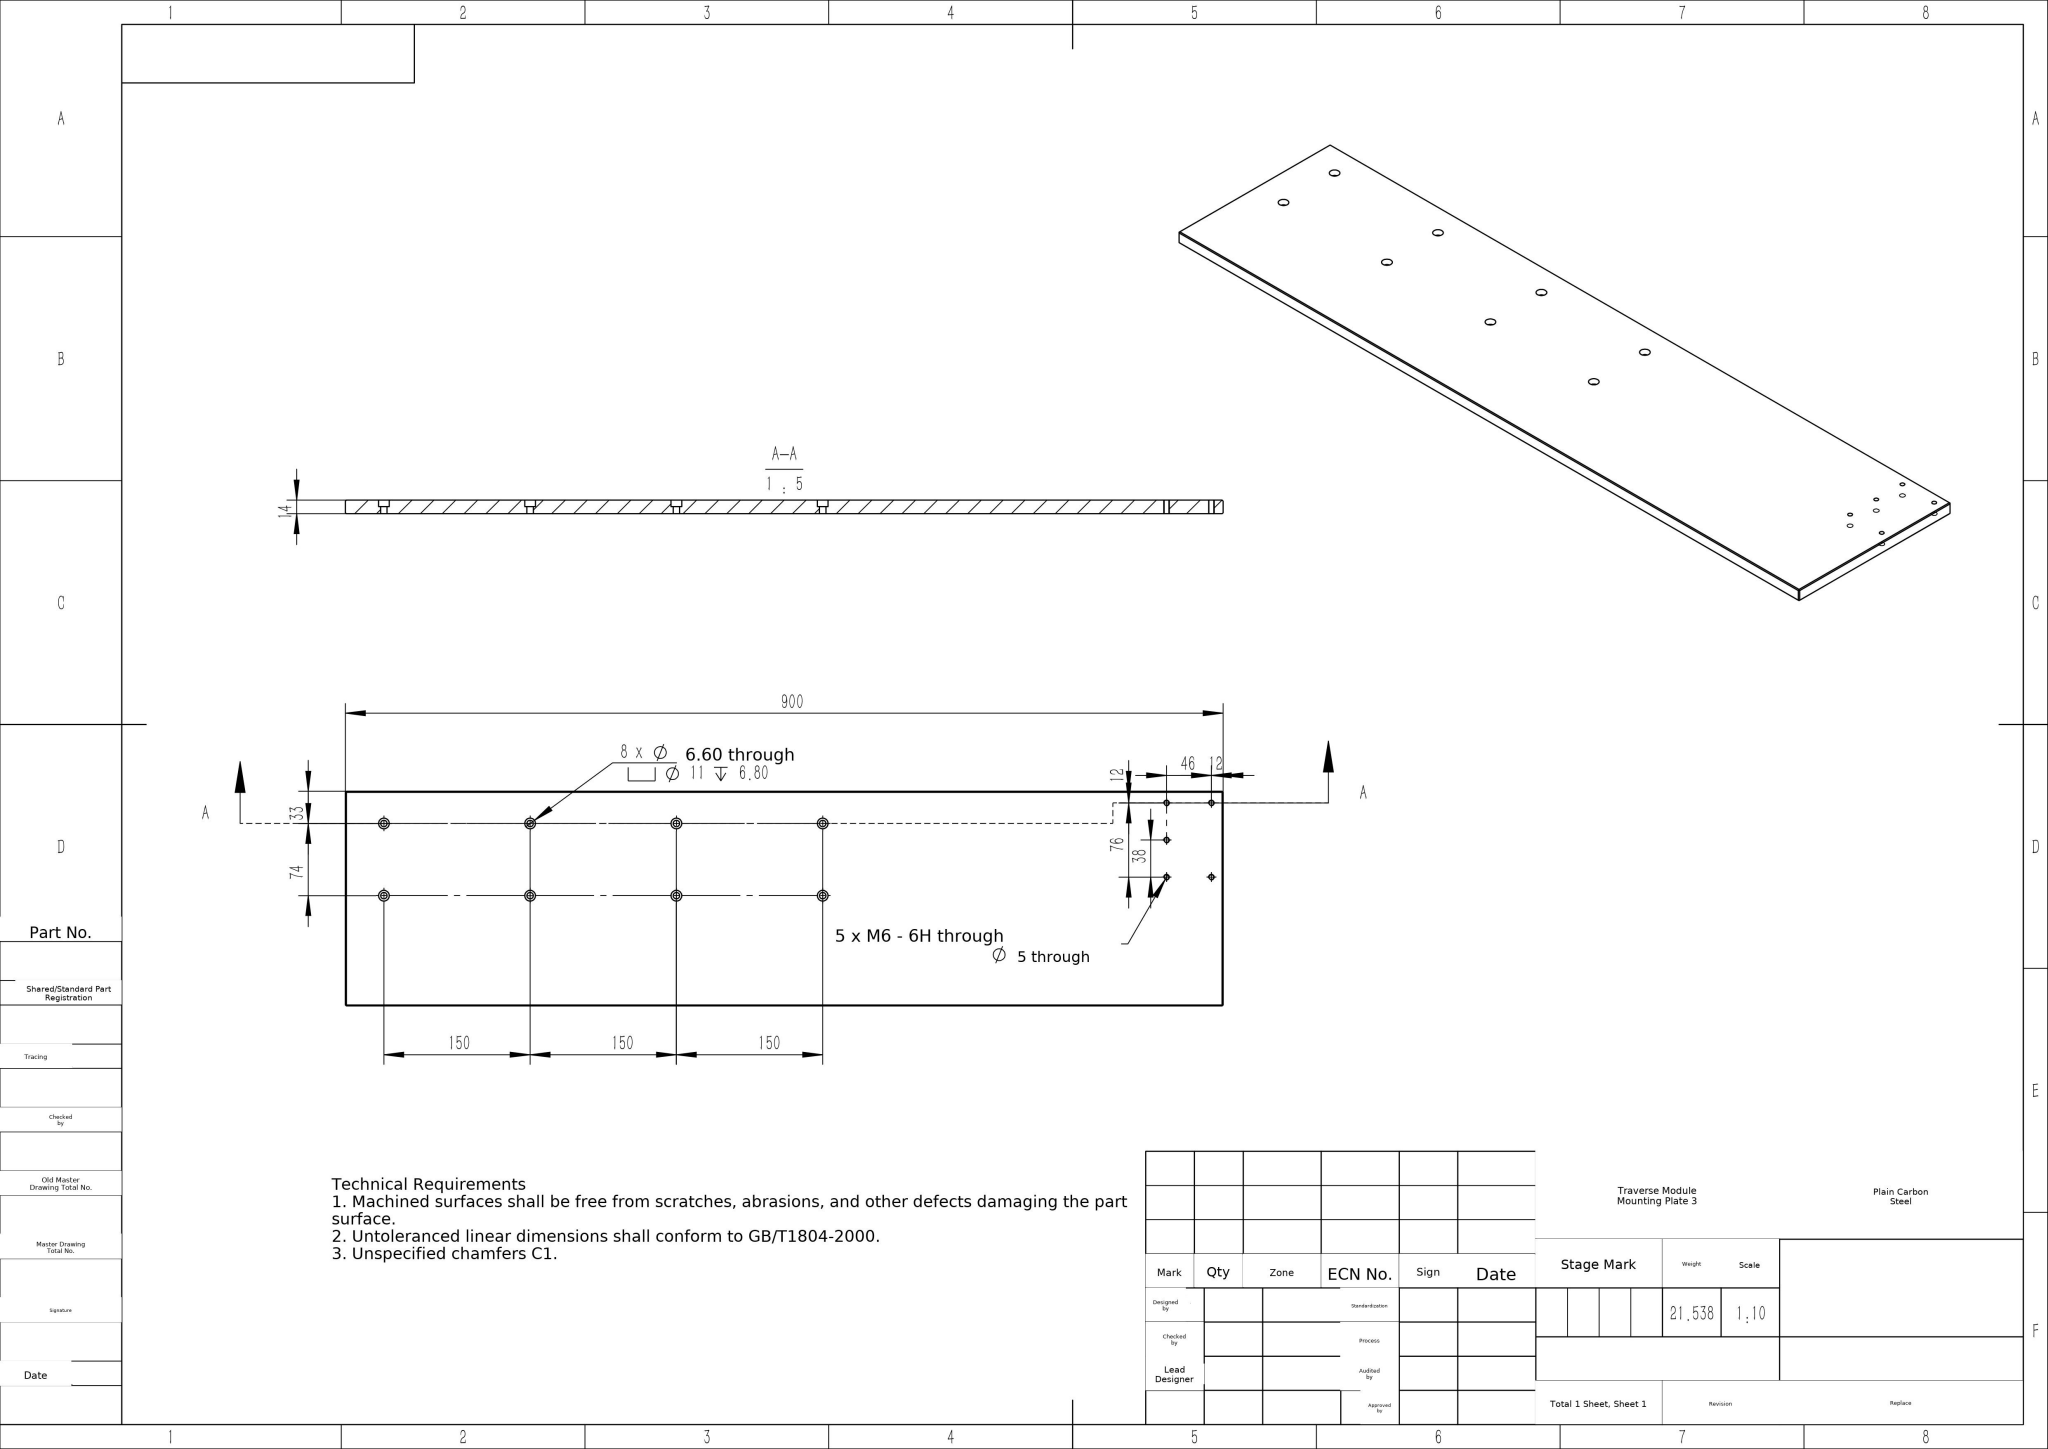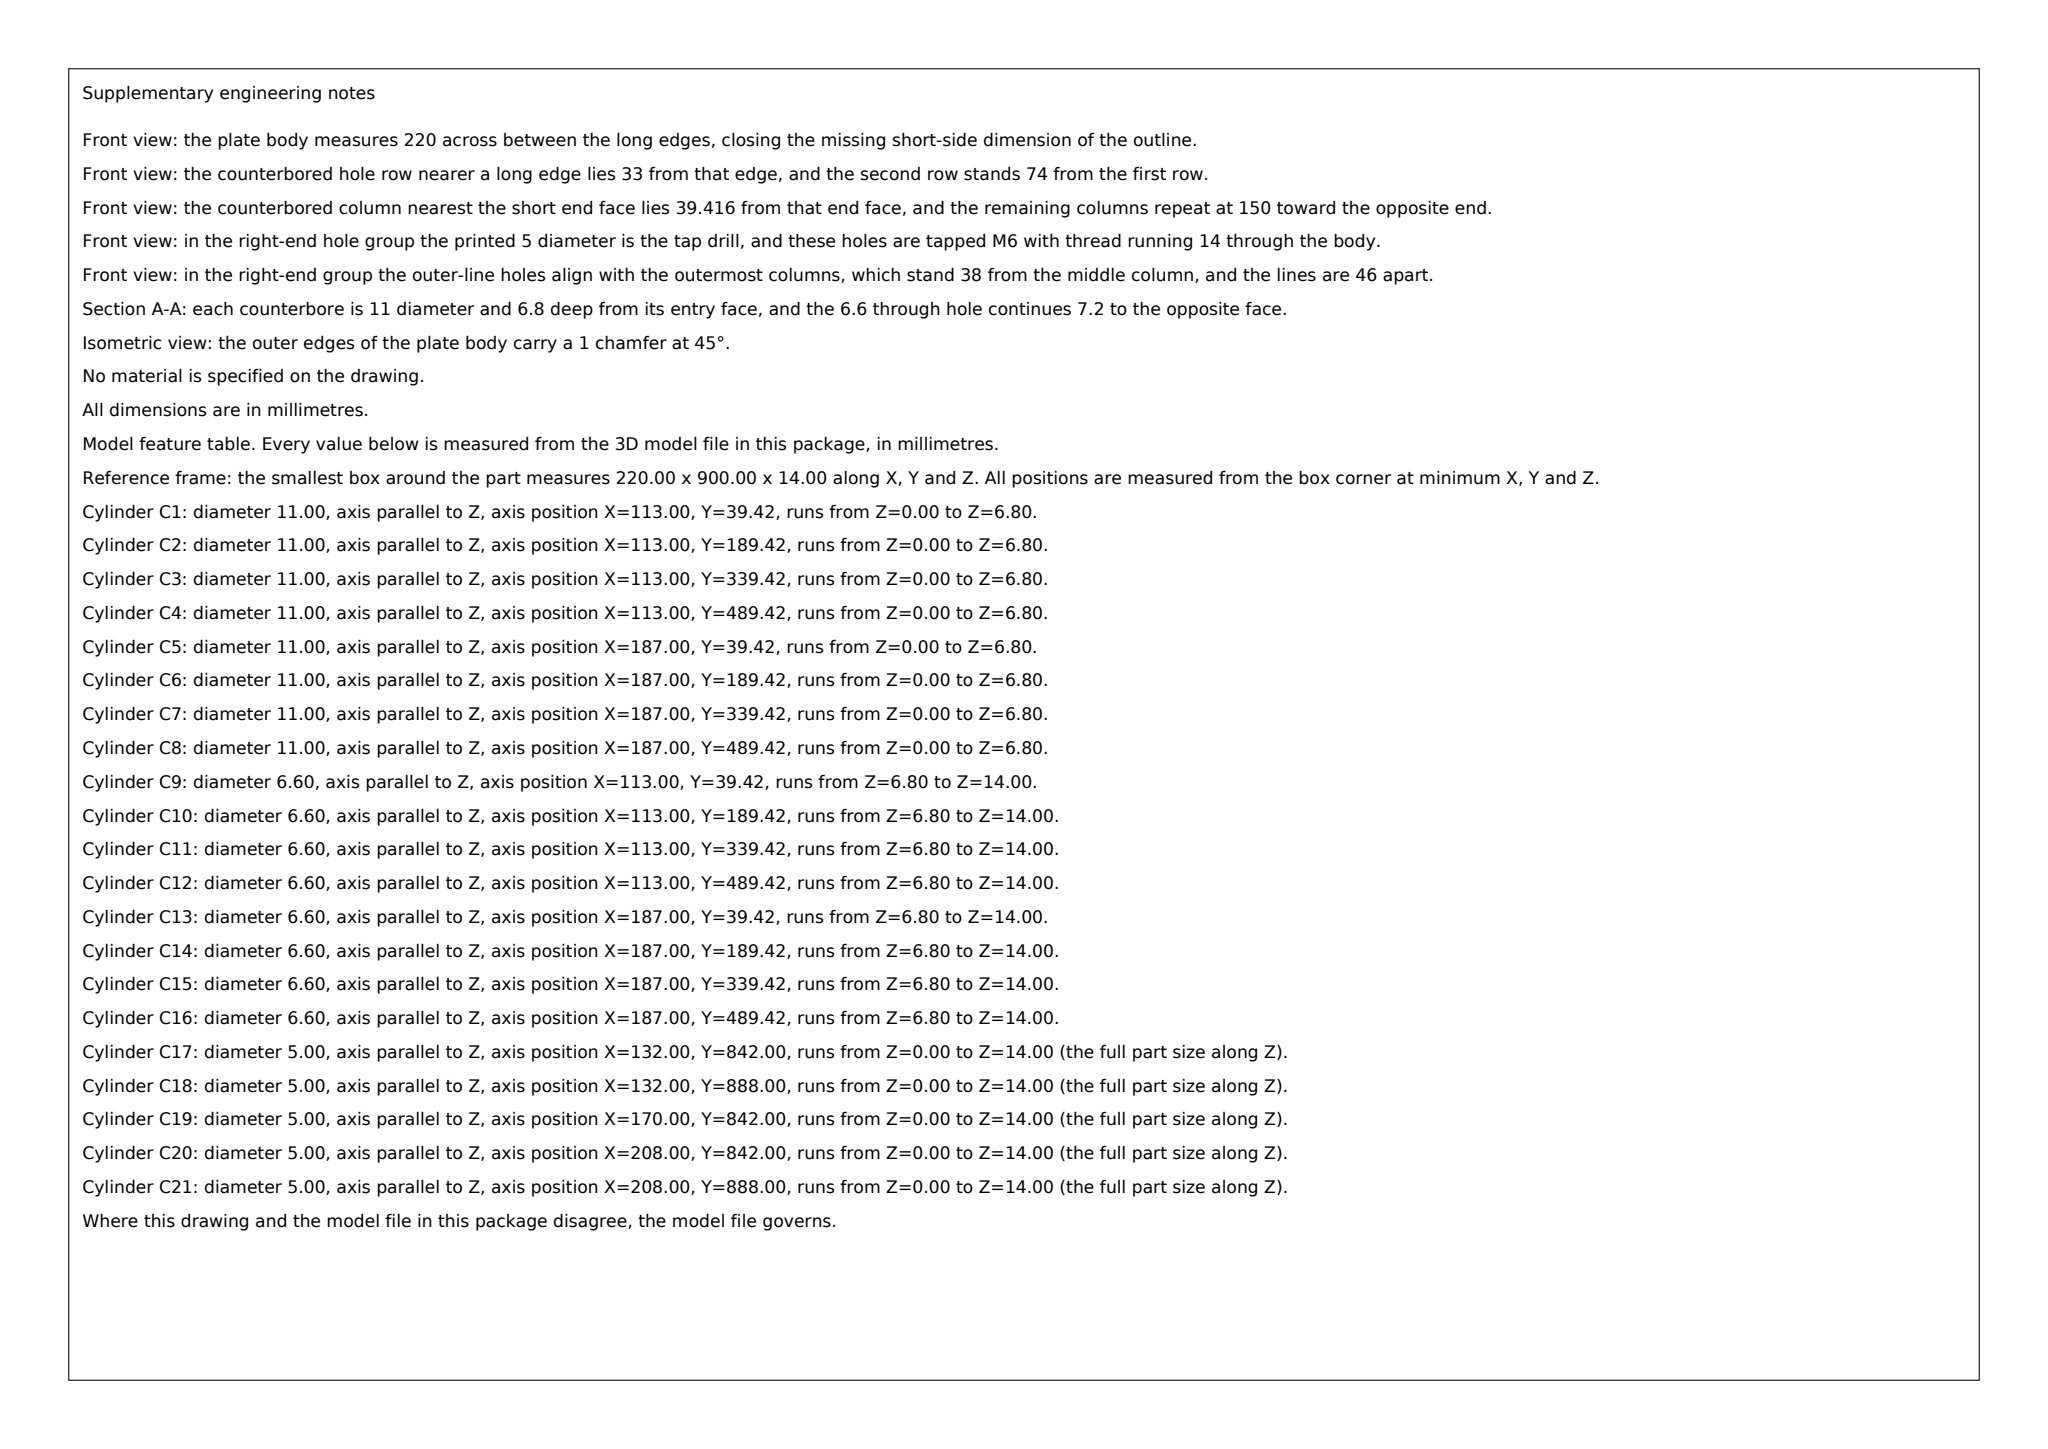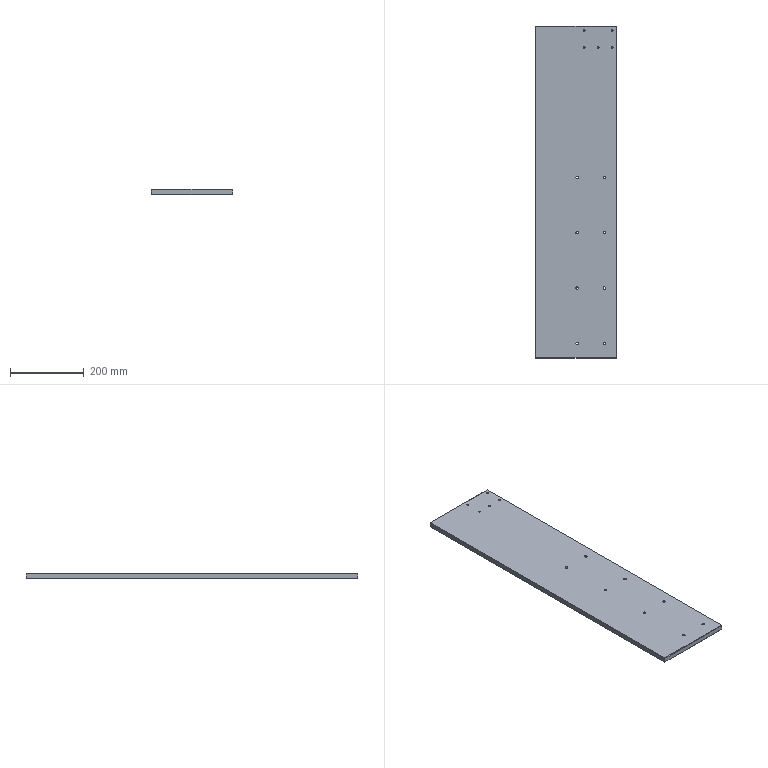Part | SolidWorks | mm | 1 solid | 76 faces | box 220 x 900 x 14 mm | volume 2761222 mm3 | cylinder 42 | plane 34 | commonest cylinder face diameters 11 x16 6.6 x16 5 x10
build123d program:
from build123d import *

# Parameters (mm, degrees)
SKETCH1_W                                       = 220
SKETCH1_H                                       = 900
BOSS_EXTRUDE1_DEPTH                             = 14
CHAMFER1_SIZE                                   = 1
M6_TAPPED_HOLE1_D                               = 5
M6_HEX_SOCKET_HEAD_CAP_SCREW_CBORE1_D           = 6.6
M6_HEX_SOCKET_HEAD_CAP_SCREW_CBORE1_CBORE_D     = 11
M6_HEX_SOCKET_HEAD_CAP_SCREW_CBORE1_CBORE_DEPTH = 6.8
LPATTERN1_COUNT                                 = 4
LPATTERN1_PITCH                                 = 150


with BuildPart() as part:
    # Sketch1 → Boss-Extrude1 (new body)
    with BuildSketch(Plane.XY):
        Rectangle(SKETCH1_W, SKETCH1_H)
    extrude(amount=BOSS_EXTRUDE1_DEPTH)

    # Chamfer1
    chamfer1_edges = [part.edges().sort_by_distance(p)[0] for p in [
        (0, 450, 14),
        (-110, 0, 14),
        (0, -450, 14),
        (-110, 0, 0),
        (0, 450, 0),
        (110, 0, 0),
        (0, -450, 0),
        (-110, -450, 7),
        (-110, 450, 7),
        (110, 450, 7),
        (110, -450, 7),
        (110, 0, 14),
    ]]
    chamfer(chamfer1_edges, length=CHAMFER1_SIZE)

    # M6 Tapped Hole1 (through all)
    with Locations(Plane.XY.offset(14)):
        with Locations((22, 438), (22, 392), (60, 392), (98, 438), (98, 392)):
            Hole(M6_TAPPED_HOLE1_D / 2)

    # M6 Hex Socket Head Cap Screw CBORE1 (through all)
    with Locations(Plane(origin=(0, 0, 0), x_dir=(-1, 0, 0), z_dir=(0, 0, -1))):
        with Locations((-77, -410.584), (-3, -410.584)):
            m6_hex_socket_head_cap_screw_cbore1 = CounterBoreHole(M6_HEX_SOCKET_HEAD_CAP_SCREW_CBORE1_D / 2, M6_HEX_SOCKET_HEAD_CAP_SCREW_CBORE1_CBORE_D / 2, M6_HEX_SOCKET_HEAD_CAP_SCREW_CBORE1_CBORE_DEPTH)

    # LPattern1: M6 Hex Socket Head Cap Screw CBORE1 ×4
    with Locations(*[(0, i * LPATTERN1_PITCH, 0) for i in range(1, LPATTERN1_COUNT)]):
        add(m6_hex_socket_head_cap_screw_cbore1, mode=Mode.SUBTRACT)


solid = part.part